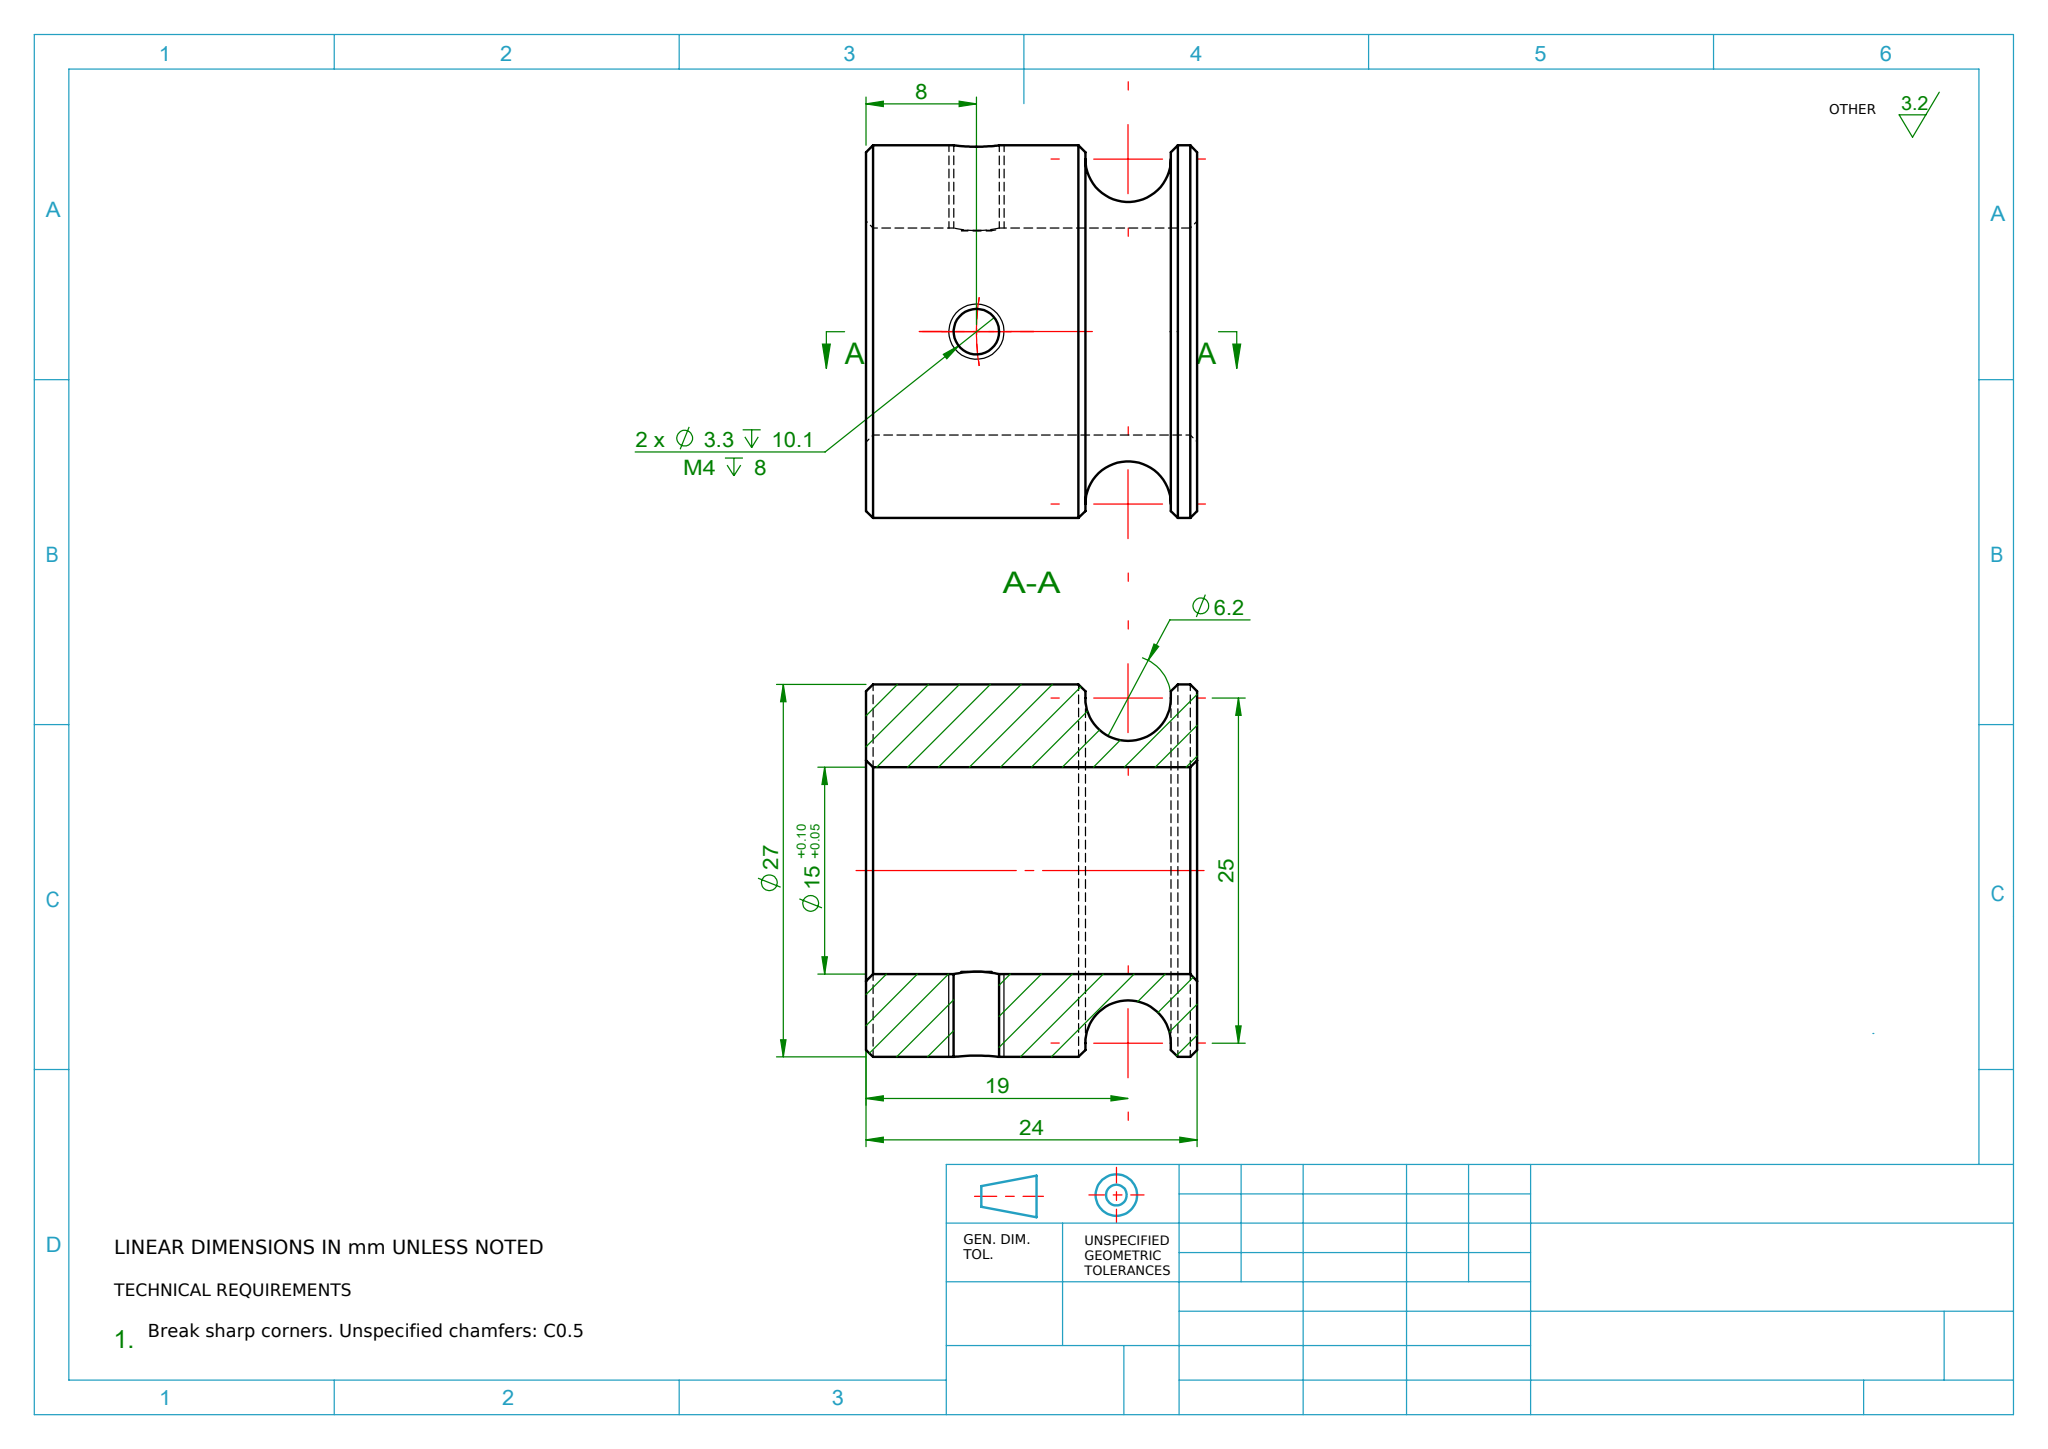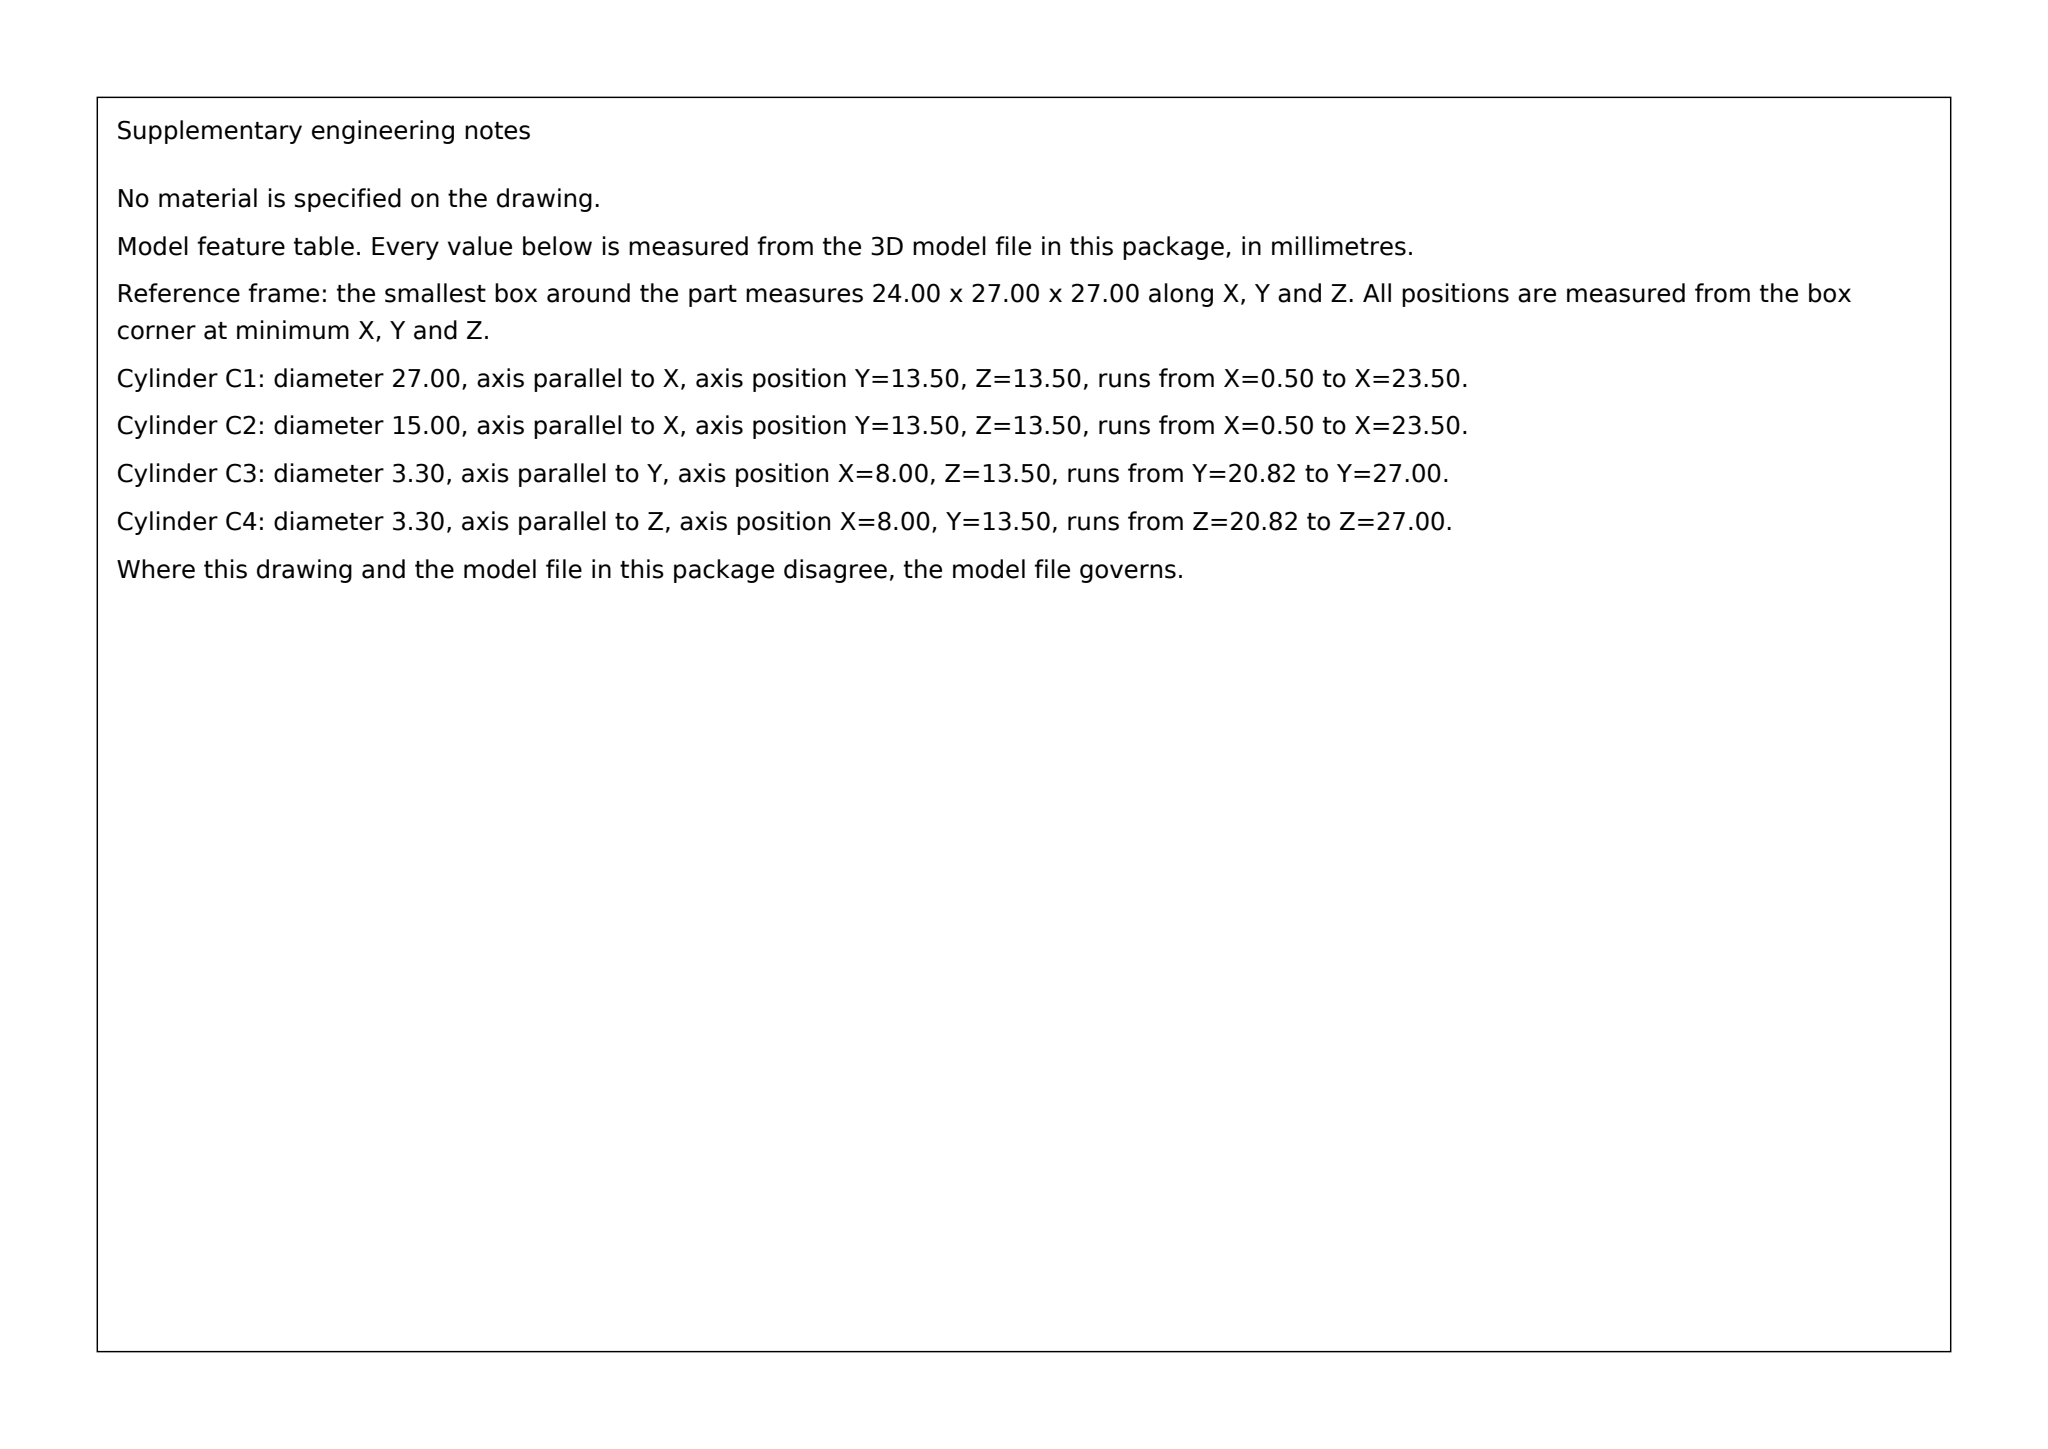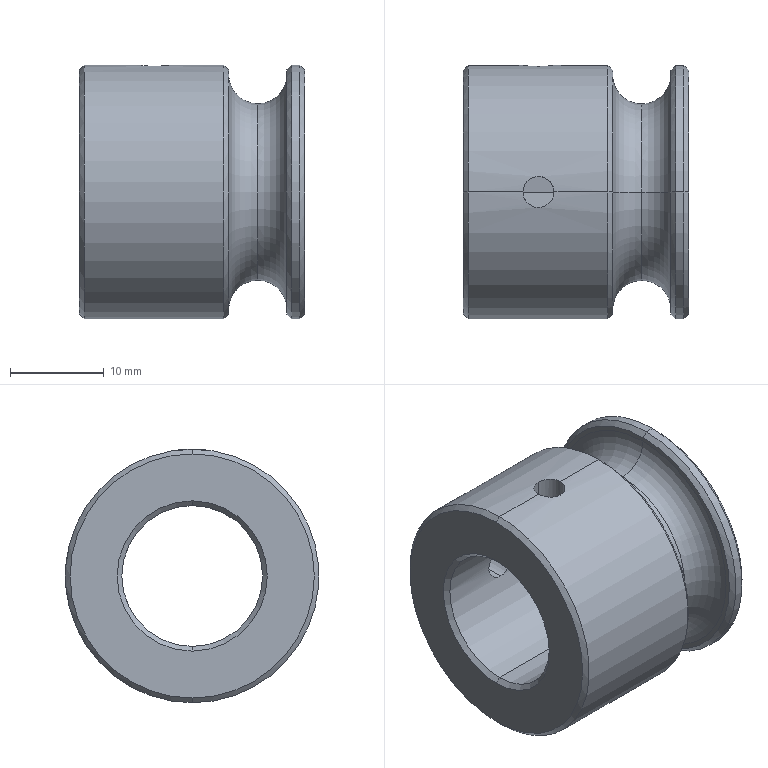Part | SolidWorks | mm | 1 solid | 30 faces | box 24 x 27 x 27 mm | volume 7776 mm3 | cone 12 | cylinder 10 | torus 4 | plane 4 | commonest cylinder face diameters 3.3 x4 27 x4 15 x2
build123d program:
from build123d import *

# Parameters (mm, degrees)
SKETCH1_R           = 13.5
SKETCH1_R_2         = 7.5
BOSS_EXTRUDE1_DEPTH = 24
CHAMFER1_SIZE       = 0.5
CIRPATTERN1_COUNT   = 2
CIRPATTERN1_ANGLE   = 90


with BuildPart() as part:
    # Sketch1 → Boss-Extrude1 (new body)
    with BuildSketch(Plane(origin=(0, 0, 0), x_dir=(0, 0, -1), z_dir=(1, 0, 0))):
        Circle(SKETCH1_R)
        Circle(SKETCH1_R_2, mode=Mode.SUBTRACT)
    extrude(amount=BOSS_EXTRUDE1_DEPTH)

    # Sketch2 → Cut-Revolve1 (revolve, cut)
    with BuildSketch(Plane.XY, mode=Mode.PRIVATE) as cut_revolve1_sk:
        with BuildLine():
            Line((15.9, 12.5), (15.9, 16.614))
            Line((15.9, 16.614), (22.1, 16.614))
            Line((22.1, 16.614), (22.1, 12.5))
            ThreePointArc((22.1, 12.5), (19, 9.4), (15.9, 12.5))
        make_face()
    revolve(cut_revolve1_sk.sketch.rotate(Axis((0, 0, 0), (1, 0, 0)), 90), axis=Axis((0, 0, 0), (1, 0, 0)), mode=Mode.SUBTRACT)

    # Chamfer1
    chamfer1_edges = [part.edges().sort_by_distance(p)[0] for p in [
        (22.1, 0, 13.5),
        (15.9, 0, 13.5),
        (0, 0, 13.5),
        (24, 0, 13.5),
        (0, 0, 7.5),
        (24, 0, 7.5),
    ]]
    chamfer(chamfer1_edges, length=CHAMFER1_SIZE)

    # Sketch4 → M4 Tapped Hole1 (revolve, cut)
    with BuildSketch(Plane(origin=(8, 13.5, 0), x_dir=(0, 0, 1), z_dir=(1, 0, 0))):
        Polygon((0, 0), (0, 11.091), (1.65, 10.1), (1.65, 0), align=None)
    m4_tapped_hole1 = revolve(axis=Axis((8, 19.85, 0), (0, -1, 0)), mode=Mode.SUBTRACT)

    # CirPattern1: M4 Tapped Hole1 ×2 about axis
    cirpattern1_axis = Axis((24, 0, 0), (1, 0, 0))
    for i in range(1, CIRPATTERN1_COUNT):
        add(m4_tapped_hole1.rotate(cirpattern1_axis, i * CIRPATTERN1_ANGLE / (CIRPATTERN1_COUNT - 1)), mode=Mode.SUBTRACT)


solid = part.part